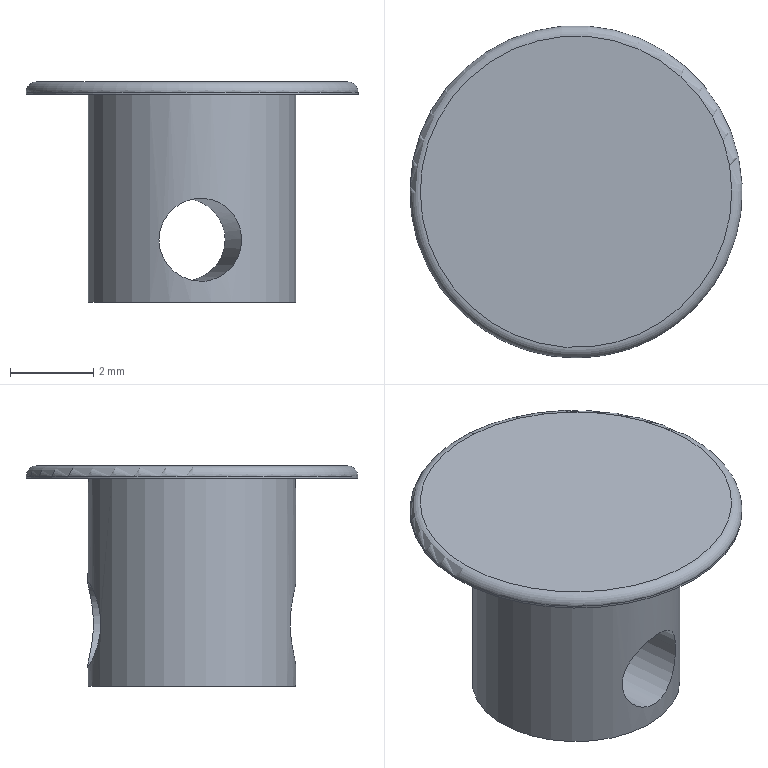Component | NX | CONNECTING_PIN | 1 solid | 7 faces | volume 98 mm3 | cylinder 3 | plane 3 | torus 1 | commonest cylinder face diameters 5 x1 8 x1 2 x1